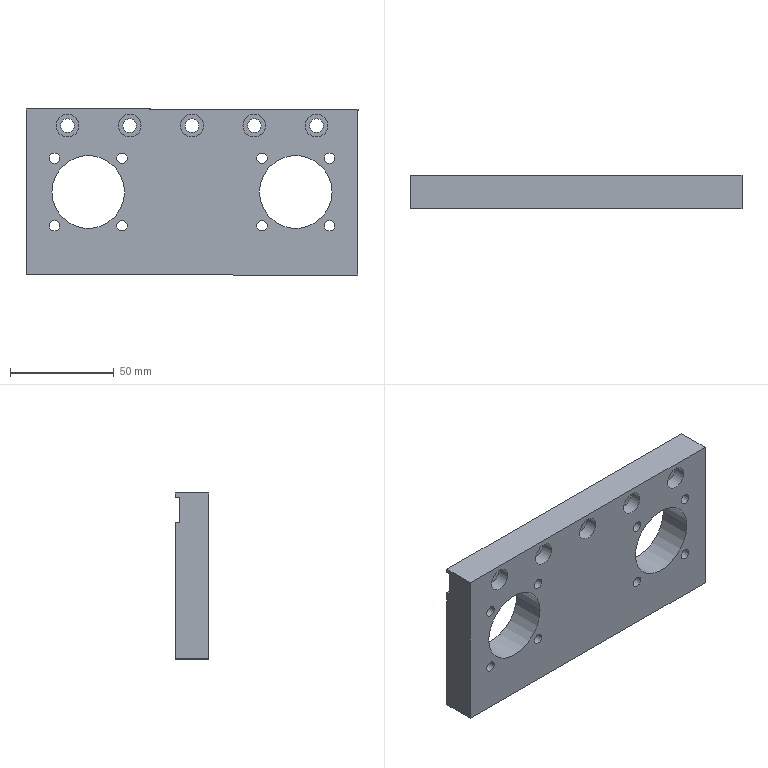Component | SolidWorks | SupportPlate_2-1 | 1 solid | 55 faces | box 160 x 16 x 80 mm | volume 163440 mm3 | cylinder 40 | plane 15 | commonest cylinder face diameters 5 x16 11 x10 6.6 x10 35 x4
build123d program:
from build123d import *

# Parameters (mm, degrees)
SKETCH1_W                                       = 160
SKETCH1_H                                       = 80
SKETCH1_R                                       = 17.5
EXTRUDE1_DEPTH                                  = 16
SKETCH2_W                                       = 160
SKETCH2_H                                       = 12
EXTRUDE2_DEPTH                                  = 2
M6_HEX_SOCKET_HEAD_CAP_SCREW_CBORE1_D           = 6.6
M6_HEX_SOCKET_HEAD_CAP_SCREW_CBORE1_CBORE_D     = 11
M6_HEX_SOCKET_HEAD_CAP_SCREW_CBORE1_CBORE_DEPTH = 6
M6_TAPPED_HOLE1_AT_2_COUNT                      = 2
M6_TAPPED_HOLE1_AT_2_PITCH                      = 46
M6_TAPPED_HOLE1_AT_3_COUNT                      = 2
M6_TAPPED_HOLE1_AT_3_PITCH                      = 32.527
M6_TAPPED_HOLE1_AT_4_COUNT                      = 2
M6_TAPPED_HOLE1_AT_4_PITCH                      = 32.527
LPATTERN1_COUNT                                 = 2
LPATTERN1_PITCH                                 = 100


with BuildPart() as part:
    # Sketch1 → Extrude1 (new body)
    with BuildSketch(Plane.XY):
        with Locations((27.803, -13.606)):
            Rectangle(SKETCH1_W, SKETCH1_H)
        with Locations((-22.197, -13.606)):
            Circle(SKETCH1_R, mode=Mode.SUBTRACT)
        with Locations((77.803, -13.606)):
            Circle(SKETCH1_R, mode=Mode.SUBTRACT)
    extrude(amount=EXTRUDE1_DEPTH)

    # Sketch2 → Extrude2 (cut)
    with BuildSketch(Plane.XY.offset(16)):
        with Locations((27.803, 18.394)):
            Rectangle(SKETCH2_W, SKETCH2_H)
    extrude(amount=-EXTRUDE2_DEPTH, mode=Mode.SUBTRACT)

    # M6 Hex Socket Head Cap Screw CBORE1 (through all)
    with Locations(Plane(origin=(0, 0, 0), x_dir=(-1, 0, 0), z_dir=(0, 0, -1))):
        with Locations((-57.803, 18.394), (-27.803, 18.394), (2.197, 18.394), (32.197, 18.394), (-87.803, 18.394)):
            CounterBoreHole(M6_HEX_SOCKET_HEAD_CAP_SCREW_CBORE1_D / 2, M6_HEX_SOCKET_HEAD_CAP_SCREW_CBORE1_CBORE_D / 2, M6_HEX_SOCKET_HEAD_CAP_SCREW_CBORE1_CBORE_DEPTH)

    # Sketch7 → M6 Tapped Hole1 (revolve, cut)
    with BuildSketch(Plane(origin=(-5.933, -29.869, 16), x_dir=(0, -1, 0), z_dir=(1, 0, 0))):
        Polygon((0, 0), (0, 18.502), (2.5, 17), (2.5, 0), align=None)
    m6_tapped_hole1 = revolve(axis=Axis((-5.933, -29.869, 22.35), (0, 0, -1)), mode=Mode.SUBTRACT)

    # M6 Tapped Hole1 at 2: M6 Tapped Hole1 ×2
    with Locations(*[Vector(-0.7071, 0.7071, 0) * (i * M6_TAPPED_HOLE1_AT_2_PITCH) for i in range(1, M6_TAPPED_HOLE1_AT_2_COUNT)]):
        add(m6_tapped_hole1, mode=Mode.SUBTRACT)

    # M6 Tapped Hole1 at 3: M6 Tapped Hole1 ×2
    with Locations(*[(0, i * M6_TAPPED_HOLE1_AT_3_PITCH, 0) for i in range(1, M6_TAPPED_HOLE1_AT_3_COUNT)]):
        add(m6_tapped_hole1, mode=Mode.SUBTRACT)

    # M6 Tapped Hole1 at 4: M6 Tapped Hole1 ×2
    with Locations(*[(-i * M6_TAPPED_HOLE1_AT_4_PITCH, 0, 0) for i in range(1, M6_TAPPED_HOLE1_AT_4_COUNT)]):
        add(m6_tapped_hole1, mode=Mode.SUBTRACT)

    # LPattern1: M6 Tapped Hole1 ×2
    with Locations(*[(i * LPATTERN1_PITCH, 0, 0) for i in range(1, LPATTERN1_COUNT)]):
        add(m6_tapped_hole1, mode=Mode.SUBTRACT)

    # LPattern1 copy 1 sketch → LPattern1 copy 1 (revolve, cut)
    with BuildSketch(Plane(origin=(61.54, 2.658, 16), x_dir=(0, -1, 0), z_dir=(1, 0, 0))):
        Polygon((0, 0), (0, 18.502), (2.5, 17), (2.5, 0), align=None)
    revolve(axis=Axis((61.54, 2.658, 22.35), (0, 0, -1)), mode=Mode.SUBTRACT)

    # LPattern1 copy 2 sketch → LPattern1 copy 2 (revolve, cut)
    with BuildSketch(Plane(origin=(94.067, 2.658, 16), x_dir=(0, -1, 0), z_dir=(1, 0, 0))):
        Polygon((0, 0), (0, 18.502), (2.5, 17), (2.5, 0), align=None)
    revolve(axis=Axis((94.067, 2.658, 22.35), (0, 0, -1)), mode=Mode.SUBTRACT)

    # LPattern1 copy 3 sketch → LPattern1 copy 3 (revolve, cut)
    with BuildSketch(Plane(origin=(61.54, -29.869, 16), x_dir=(0, -1, 0), z_dir=(1, 0, 0))):
        Polygon((0, 0), (0, 18.502), (2.5, 17), (2.5, 0), align=None)
    revolve(axis=Axis((61.54, -29.869, 22.35), (0, 0, -1)), mode=Mode.SUBTRACT)


solid = part.part

# Placed as in the assembly
solid = solid.moved(Location((-164.817, 536.983, -162.61), (-90, 0, 180)))